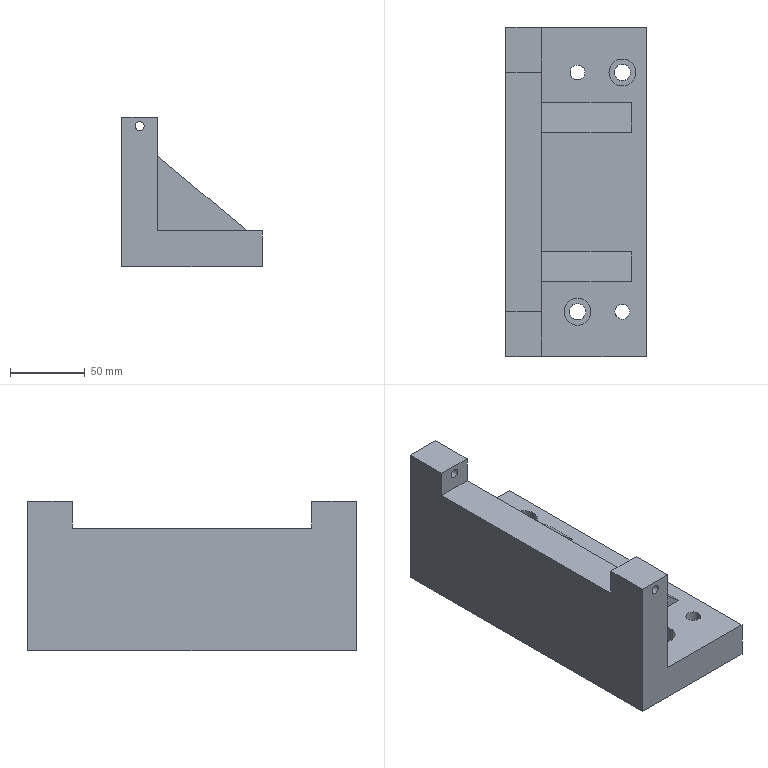Component | NX | ANGLE_BRACKET | 1 solid | 28 faces | volume 875008 mm3 | plane 20 | cylinder 8 | commonest cylinder face diameters 11 x2 18 x2 10 x2 6 x2